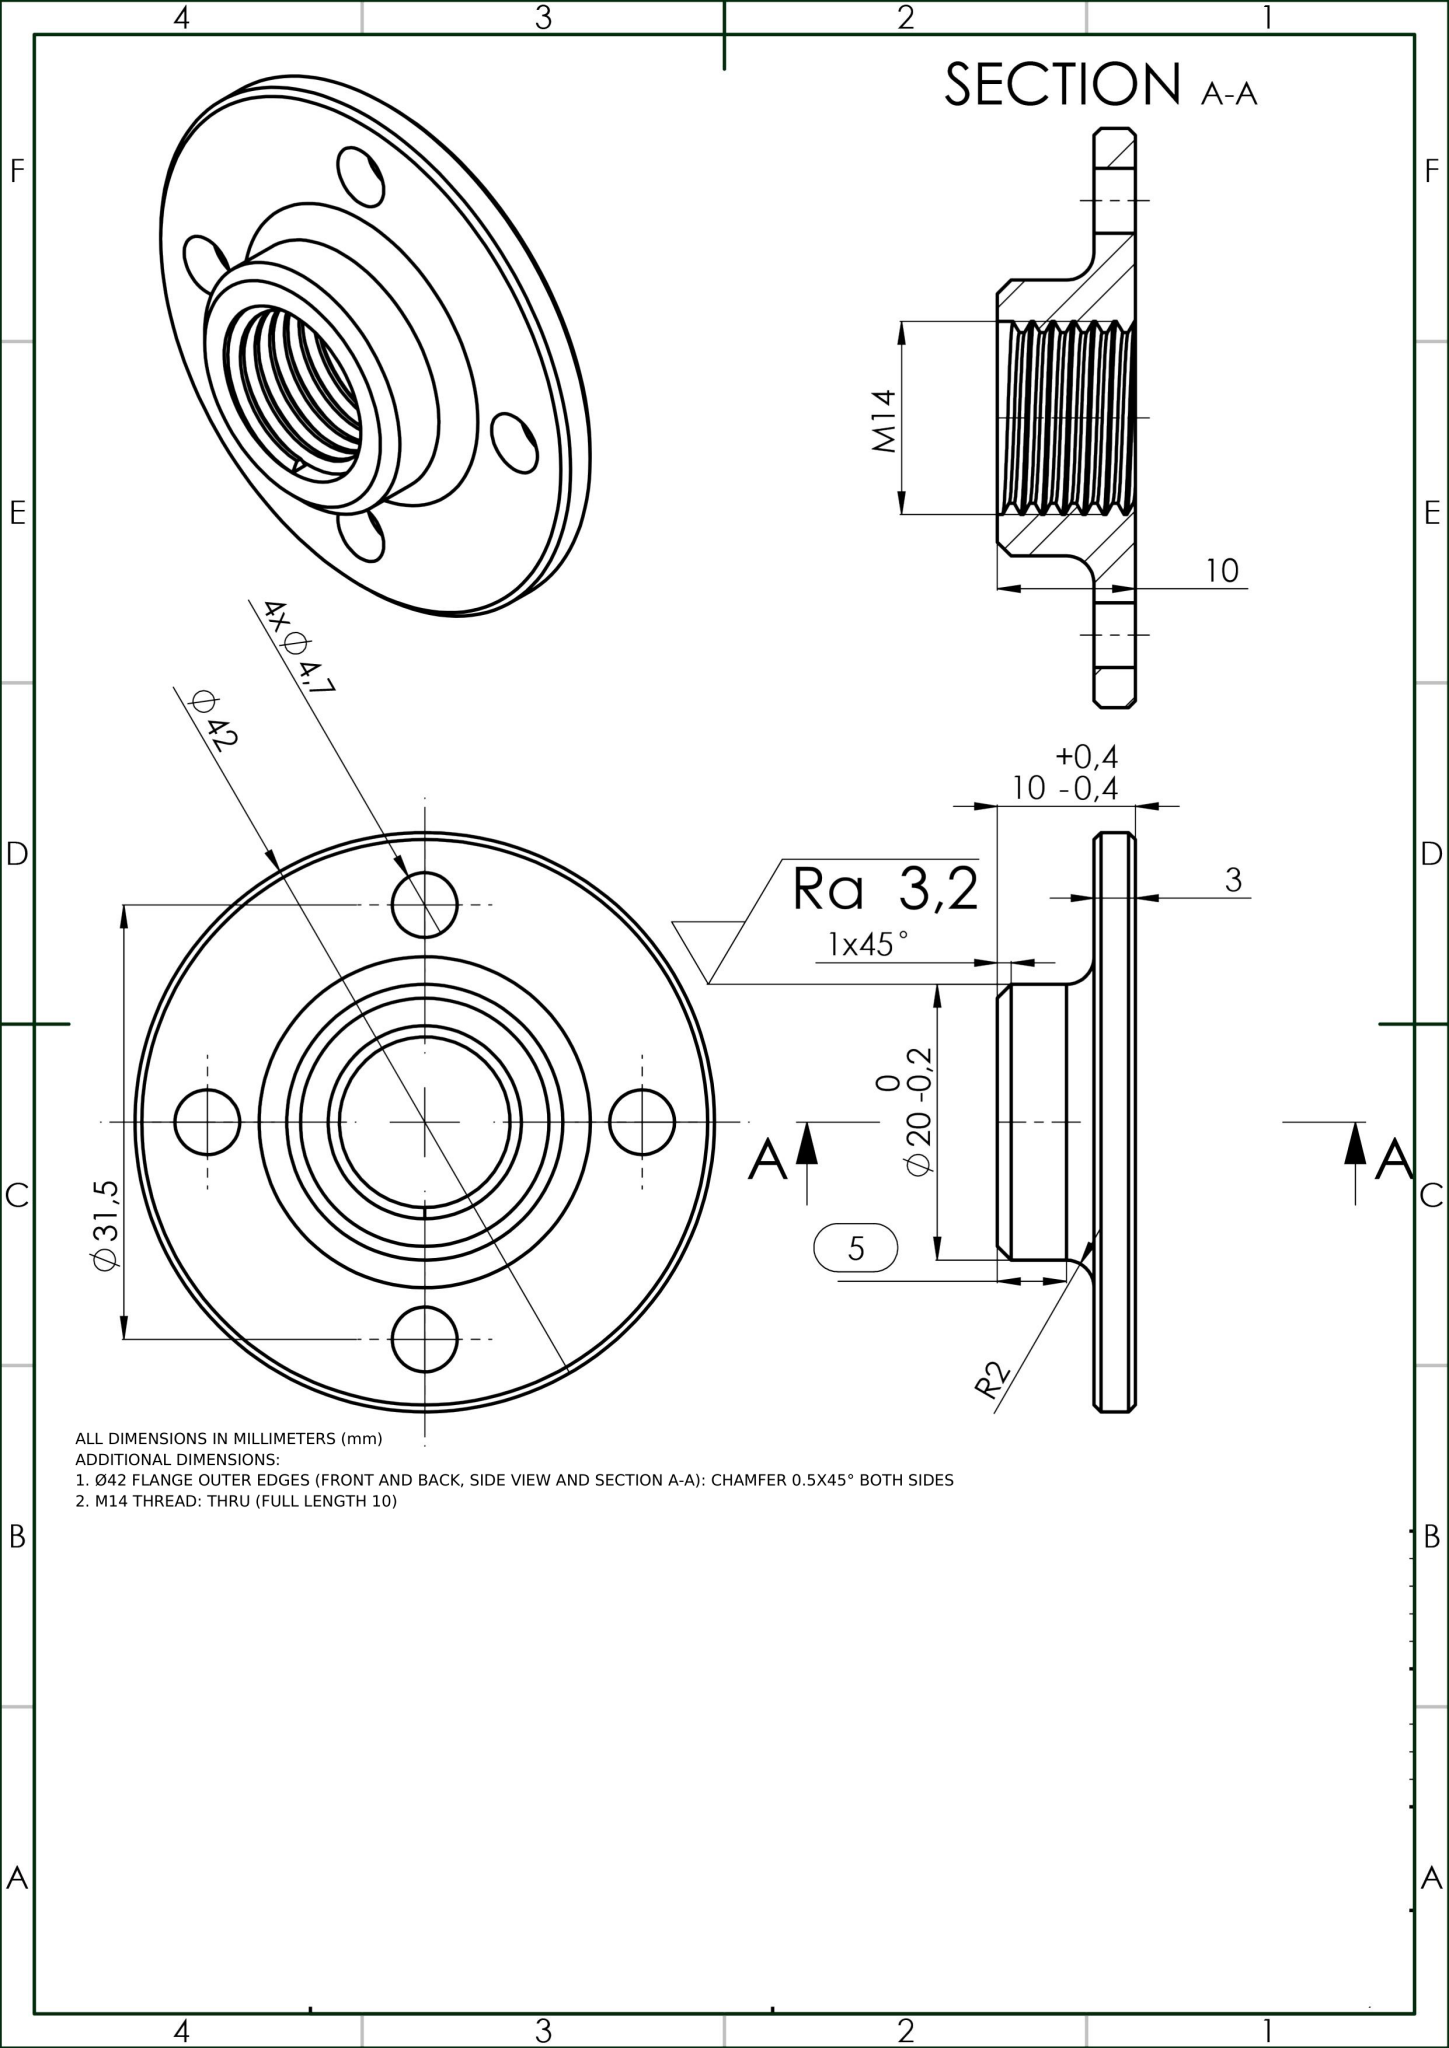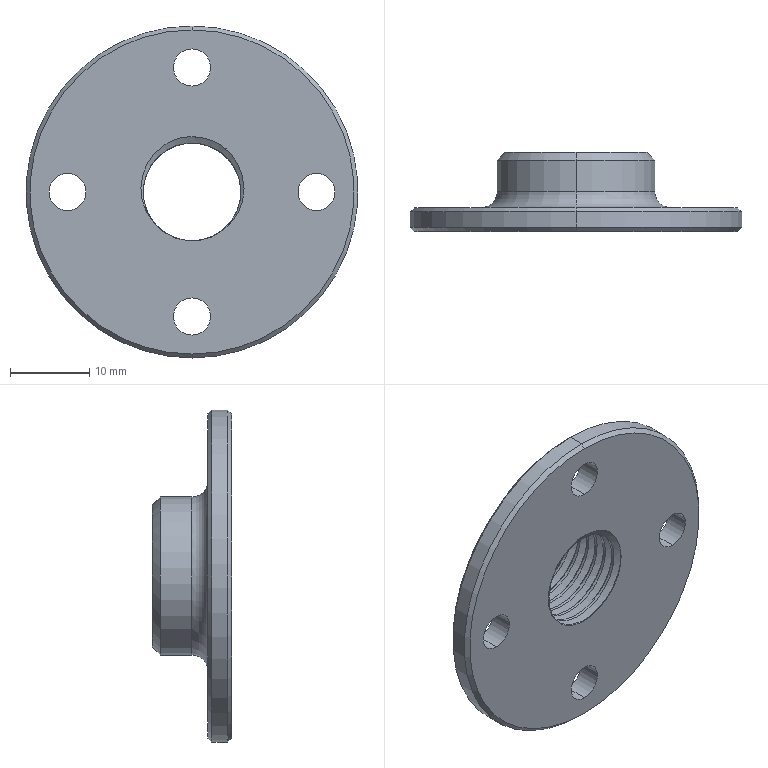Part | NX | mm | 1 solid | 42 faces | box 42 x 10 x 42 mm | volume 4780 mm3 | cylinder 27 | cone 6 | plane 4 | spline 3 | torus 2 | commonest cylinder face diameters 14 x15 4.7 x8 20 x2 42 x2